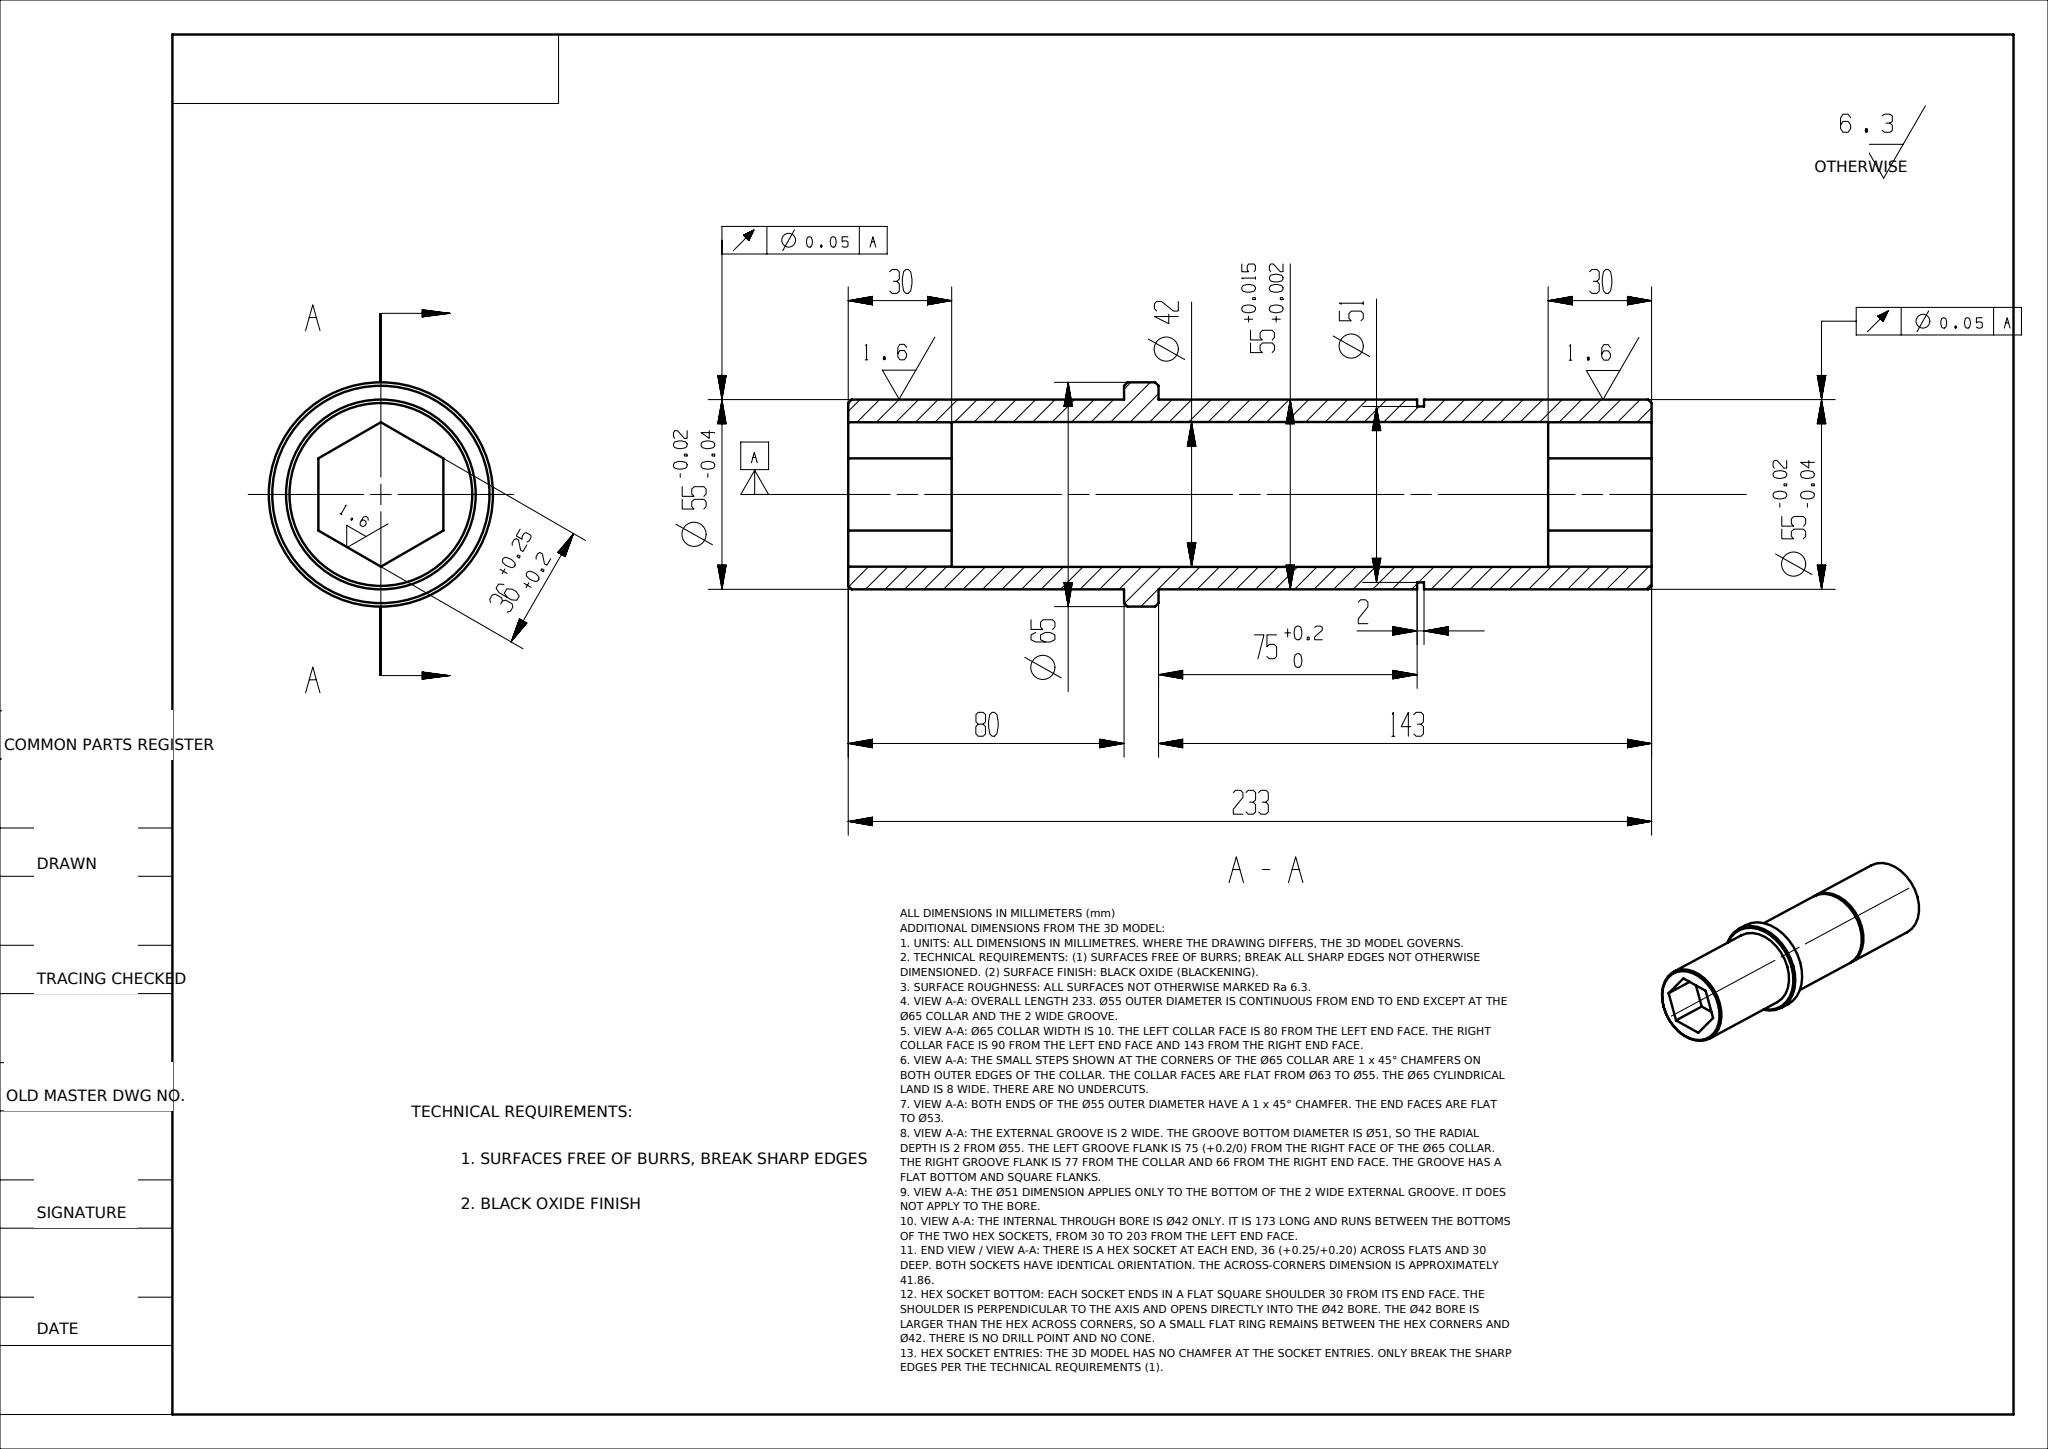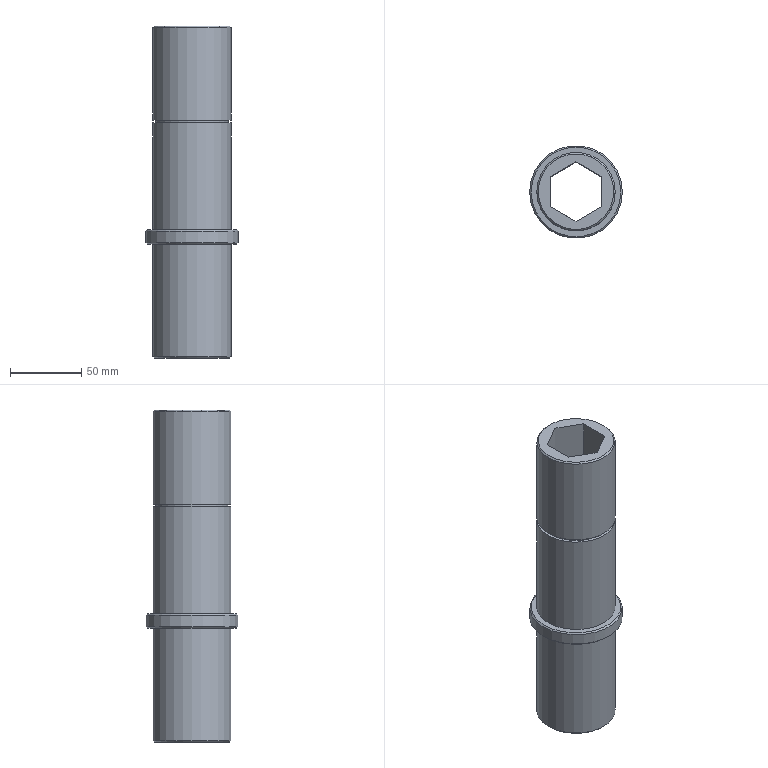Part | NX | mm | 1 solid | 30 faces | box 65 x 65 x 233 mm | volume 253992 mm3 | plane 20 | cylinder 6 | cone 4 | commonest cylinder face diameters 55 x3 65 x1 51 x1 42 x1
STEP:
#1=CARTESIAN_POINT('',(0.,0.,0.));
#2=DIRECTION('',(0.,0.,1.));
#3=DIRECTION('',(1.,0.,0.));
#4=AXIS2_PLACEMENT_3D('',#1,#2,#3);
#5=(LENGTH_UNIT()NAMED_UNIT(*)SI_UNIT(.MILLI.,.METRE.));
#6=UNCERTAINTY_MEASURE_WITH_UNIT(LENGTH_MEASURE(0.00002),#5,'','');
#7=(NAMED_UNIT(*)PLANE_ANGLE_UNIT()SI_UNIT($,.RADIAN.));
#8=PLANE_ANGLE_MEASURE_WITH_UNIT(PLANE_ANGLE_MEASURE(0.01745),#7);
#9=DIMENSIONAL_EXPONENTS(0.,0.,0.,0.,0.,0.,0.);
#10=(CONVERSION_BASED_UNIT('',#8)NAMED_UNIT(#9)PLANE_ANGLE_UNIT());
#11=(NAMED_UNIT(*)SI_UNIT($,.STERADIAN.)SOLID_ANGLE_UNIT());
#12=(GEOMETRIC_REPRESENTATION_CONTEXT(3)GLOBAL_UNCERTAINTY_ASSIGNED_CONTEXT((#6))GLOBAL_UNIT_ASSIGNED_CONTEXT((#5,#10,#11))REPRESENTATION_CONTEXT('',''));
#13=SHAPE_REPRESENTATION('',(#4),#12);
#14=CARTESIAN_POINT('',(-26.5,0.,20.));
#15=VERTEX_POINT('',#14);
#16=CARTESIAN_POINT('',(0.,0.,20.));
#17=DIRECTION('',(0.,0.,-1.));
#18=DIRECTION('',(-1.,0.,0.));
#19=AXIS2_PLACEMENT_3D('',#16,#17,#18);
#20=CIRCLE('',#19,26.5);
#21=EDGE_CURVE('',#15,#15,#20,.T.);
#22=ORIENTED_EDGE('',*,*,#21,.T.);
#23=EDGE_LOOP('',(#22));
#24=FACE_BOUND('',#23,.T.);
#25=CARTESIAN_POINT('',(-0.,20.929,20.));
#26=VERTEX_POINT('',#25);
#27=CARTESIAN_POINT('',(-18.125,10.464,20.));
#28=VERTEX_POINT('',#27);
#29=CARTESIAN_POINT('',(-9.063,15.697,20.));
#30=DIRECTION('',(-0.866,-0.5,0.));
#31=VECTOR('',#30,1.);
#32=LINE('',#29,#31);
#33=EDGE_CURVE('',#26,#28,#32,.T.);
#34=ORIENTED_EDGE('',*,*,#33,.T.);
#35=CARTESIAN_POINT('',(-18.125,-10.464,20.));
#36=VERTEX_POINT('',#35);
#37=CARTESIAN_POINT('',(-18.125,0.,20.));
#38=DIRECTION('',(0.,-1.,0.));
#39=VECTOR('',#38,1.);
#40=LINE('',#37,#39);
#41=EDGE_CURVE('',#28,#36,#40,.T.);
#42=ORIENTED_EDGE('',*,*,#41,.T.);
#43=CARTESIAN_POINT('',(0.,-20.929,20.));
#44=VERTEX_POINT('',#43);
#45=CARTESIAN_POINT('',(-9.062,-15.697,20.));
#46=DIRECTION('',(0.866,-0.5,0.));
#47=VECTOR('',#46,1.);
#48=LINE('',#45,#47);
#49=EDGE_CURVE('',#36,#44,#48,.T.);
#50=ORIENTED_EDGE('',*,*,#49,.T.);
#51=CARTESIAN_POINT('',(18.125,-10.464,20.));
#52=VERTEX_POINT('',#51);
#53=CARTESIAN_POINT('',(9.063,-15.697,20.));
#54=DIRECTION('',(0.866,0.5,0.));
#55=VECTOR('',#54,1.);
#56=LINE('',#53,#55);
#57=EDGE_CURVE('',#44,#52,#56,.T.);
#58=ORIENTED_EDGE('',*,*,#57,.T.);
#59=CARTESIAN_POINT('',(18.125,10.464,20.));
#60=VERTEX_POINT('',#59);
#61=CARTESIAN_POINT('',(18.125,0.,20.));
#62=DIRECTION('',(0.,1.,0.));
#63=VECTOR('',#62,1.);
#64=LINE('',#61,#63);
#65=EDGE_CURVE('',#52,#60,#64,.T.);
#66=ORIENTED_EDGE('',*,*,#65,.T.);
#67=CARTESIAN_POINT('',(9.062,15.697,20.));
#68=DIRECTION('',(-0.866,0.5,0.));
#69=VECTOR('',#68,1.);
#70=LINE('',#67,#69);
#71=EDGE_CURVE('',#60,#26,#70,.T.);
#72=ORIENTED_EDGE('',*,*,#71,.T.);
#73=EDGE_LOOP('',(#34,#42,#50,#58,#66,#72));
#74=FACE_BOUND('',#73,.T.);
#75=CARTESIAN_POINT('',(0.,0.,20.));
#76=DIRECTION('',(0.,0.,-1.));
#77=DIRECTION('',(-1.,0.,0.));
#78=AXIS2_PLACEMENT_3D('',#75,#76,#77);
#79=PLANE('',#78);
#80=ADVANCED_FACE('',(#24,#74),#79,.T.);
#81=CARTESIAN_POINT('',(26.5,0.,253.));
#82=VERTEX_POINT('',#81);
#83=CARTESIAN_POINT('',(0.,0.,253.));
#84=DIRECTION('',(0.,0.,1.));
#85=DIRECTION('',(1.,0.,0.));
#86=AXIS2_PLACEMENT_3D('',#83,#84,#85);
#87=CIRCLE('',#86,26.5);
#88=EDGE_CURVE('',#82,#82,#87,.T.);
#89=ORIENTED_EDGE('',*,*,#88,.T.);
#90=EDGE_LOOP('',(#89));
#91=FACE_BOUND('',#90,.T.);
#92=CARTESIAN_POINT('',(0.,-20.929,253.));
#93=VERTEX_POINT('',#92);
#94=CARTESIAN_POINT('',(-18.125,-10.464,253.));
#95=VERTEX_POINT('',#94);
#96=CARTESIAN_POINT('',(-9.062,-15.697,253.));
#97=DIRECTION('',(-0.866,0.5,0.));
#98=VECTOR('',#97,1.);
#99=LINE('',#96,#98);
#100=EDGE_CURVE('',#93,#95,#99,.T.);
#101=ORIENTED_EDGE('',*,*,#100,.T.);
#102=CARTESIAN_POINT('',(-18.125,10.464,253.));
#103=VERTEX_POINT('',#102);
#104=CARTESIAN_POINT('',(-18.125,0.,253.));
#105=DIRECTION('',(0.,1.,0.));
#106=VECTOR('',#105,1.);
#107=LINE('',#104,#106);
#108=EDGE_CURVE('',#95,#103,#107,.T.);
#109=ORIENTED_EDGE('',*,*,#108,.T.);
#110=CARTESIAN_POINT('',(-0.,20.929,253.));
#111=VERTEX_POINT('',#110);
#112=CARTESIAN_POINT('',(-9.063,15.697,253.));
#113=DIRECTION('',(0.866,0.5,0.));
#114=VECTOR('',#113,1.);
#115=LINE('',#112,#114);
#116=EDGE_CURVE('',#103,#111,#115,.T.);
#117=ORIENTED_EDGE('',*,*,#116,.T.);
#118=CARTESIAN_POINT('',(18.125,10.464,253.));
#119=VERTEX_POINT('',#118);
#120=CARTESIAN_POINT('',(9.062,15.697,253.));
#121=DIRECTION('',(0.866,-0.5,0.));
#122=VECTOR('',#121,1.);
#123=LINE('',#120,#122);
#124=EDGE_CURVE('',#111,#119,#123,.T.);
#125=ORIENTED_EDGE('',*,*,#124,.T.);
#126=CARTESIAN_POINT('',(18.125,-10.464,253.));
#127=VERTEX_POINT('',#126);
#128=CARTESIAN_POINT('',(18.125,0.,253.));
#129=DIRECTION('',(0.,-1.,0.));
#130=VECTOR('',#129,1.);
#131=LINE('',#128,#130);
#132=EDGE_CURVE('',#119,#127,#131,.T.);
#133=ORIENTED_EDGE('',*,*,#132,.T.);
#134=CARTESIAN_POINT('',(9.063,-15.697,253.));
#135=DIRECTION('',(-0.866,-0.5,0.));
#136=VECTOR('',#135,1.);
#137=LINE('',#134,#136);
#138=EDGE_CURVE('',#127,#93,#137,.T.);
#139=ORIENTED_EDGE('',*,*,#138,.T.);
#140=EDGE_LOOP('',(#101,#109,#117,#125,#133,#139));
#141=FACE_BOUND('',#140,.T.);
#142=CARTESIAN_POINT('',(0.,0.,253.));
#143=DIRECTION('',(0.,0.,1.));
#144=DIRECTION('',(1.,0.,0.));
#145=AXIS2_PLACEMENT_3D('',#142,#143,#144);
#146=PLANE('',#145);
#147=ADVANCED_FACE('',(#91,#141),#146,.T.);
#148=CARTESIAN_POINT('',(27.5,0.,110.));
#149=VERTEX_POINT('',#148);
#150=CARTESIAN_POINT('',(0.,0.,110.));
#151=DIRECTION('',(0.,0.,-1.));
#152=DIRECTION('',(1.,0.,0.));
#153=AXIS2_PLACEMENT_3D('',#150,#151,#152);
#154=CIRCLE('',#153,27.5);
#155=EDGE_CURVE('',#149,#149,#154,.T.);
#156=ORIENTED_EDGE('',*,*,#155,.F.);
#157=EDGE_LOOP('',(#156));
#158=FACE_BOUND('',#157,.T.);
#159=CARTESIAN_POINT('',(27.5,0.,185.));
#160=VERTEX_POINT('',#159);
#161=CARTESIAN_POINT('',(0.,0.,185.));
#162=DIRECTION('',(0.,0.,-1.));
#163=DIRECTION('',(1.,0.,0.));
#164=AXIS2_PLACEMENT_3D('',#161,#162,#163);
#165=CIRCLE('',#164,27.5);
#166=EDGE_CURVE('',#160,#160,#165,.T.);
#167=ORIENTED_EDGE('',*,*,#166,.T.);
#168=EDGE_LOOP('',(#167));
#169=FACE_BOUND('',#168,.T.);
#170=CARTESIAN_POINT('',(0.,0.,0.));
#171=DIRECTION('',(0.,0.,1.));
#172=DIRECTION('',(1.,0.,0.));
#173=AXIS2_PLACEMENT_3D('',#170,#171,#172);
#174=CYLINDRICAL_SURFACE('',#173,27.5);
#175=ADVANCED_FACE('',(#158,#169),#174,.T.);
#176=CARTESIAN_POINT('',(32.5,0.,109.));
#177=VERTEX_POINT('',#176);
#178=CARTESIAN_POINT('',(0.,0.,109.));
#179=DIRECTION('',(0.,0.,-1.));
#180=DIRECTION('',(1.,0.,0.));
#181=AXIS2_PLACEMENT_3D('',#178,#179,#180);
#182=CIRCLE('',#181,32.5);
#183=EDGE_CURVE('',#177,#177,#182,.T.);
#184=ORIENTED_EDGE('',*,*,#183,.T.);
#185=EDGE_LOOP('',(#184));
#186=FACE_BOUND('',#185,.T.);
#187=CARTESIAN_POINT('',(32.5,0.,101.));
#188=VERTEX_POINT('',#187);
#189=CARTESIAN_POINT('',(0.,0.,101.));
#190=DIRECTION('',(0.,0.,1.));
#191=DIRECTION('',(1.,0.,0.));
#192=AXIS2_PLACEMENT_3D('',#189,#190,#191);
#193=CIRCLE('',#192,32.5);
#194=EDGE_CURVE('',#188,#188,#193,.T.);
#195=ORIENTED_EDGE('',*,*,#194,.T.);
#196=EDGE_LOOP('',(#195));
#197=FACE_BOUND('',#196,.T.);
#198=CARTESIAN_POINT('',(0.,0.,110.));
#199=DIRECTION('',(0.,0.,-1.));
#200=DIRECTION('',(-1.,0.,0.));
#201=AXIS2_PLACEMENT_3D('',#198,#199,#200);
#202=CYLINDRICAL_SURFACE('',#201,32.5);
#203=ADVANCED_FACE('',(#186,#197),#202,.T.);
#204=CARTESIAN_POINT('',(31.5,0.,110.));
#205=VERTEX_POINT('',#204);
#206=CARTESIAN_POINT('',(0.,0.,110.));
#207=DIRECTION('',(0.,0.,1.));
#208=DIRECTION('',(1.,0.,0.));
#209=AXIS2_PLACEMENT_3D('',#206,#207,#208);
#210=CIRCLE('',#209,31.5);
#211=EDGE_CURVE('',#205,#205,#210,.T.);
#212=ORIENTED_EDGE('',*,*,#211,.T.);
#213=EDGE_LOOP('',(#212));
#214=FACE_BOUND('',#213,.T.);
#215=ORIENTED_EDGE('',*,*,#155,.T.);
#216=EDGE_LOOP('',(#215));
#217=FACE_BOUND('',#216,.T.);
#218=CARTESIAN_POINT('',(0.,0.,110.));
#219=DIRECTION('',(0.,0.,1.));
#220=DIRECTION('',(1.,0.,0.));
#221=AXIS2_PLACEMENT_3D('',#218,#219,#220);
#222=PLANE('',#221);
#223=ADVANCED_FACE('',(#214,#217),#222,.T.);
#224=CARTESIAN_POINT('',(31.5,0.,100.));
#225=VERTEX_POINT('',#224);
#226=CARTESIAN_POINT('',(0.,0.,100.));
#227=DIRECTION('',(0.,0.,-1.));
#228=DIRECTION('',(1.,0.,0.));
#229=AXIS2_PLACEMENT_3D('',#226,#227,#228);
#230=CIRCLE('',#229,31.5);
#231=EDGE_CURVE('',#225,#225,#230,.T.);
#232=ORIENTED_EDGE('',*,*,#231,.T.);
#233=EDGE_LOOP('',(#232));
#234=FACE_BOUND('',#233,.T.);
#235=CARTESIAN_POINT('',(27.5,0.,100.));
#236=VERTEX_POINT('',#235);
#237=CARTESIAN_POINT('',(0.,0.,100.));
#238=DIRECTION('',(0.,0.,-1.));
#239=DIRECTION('',(1.,0.,0.));
#240=AXIS2_PLACEMENT_3D('',#237,#238,#239);
#241=CIRCLE('',#240,27.5);
#242=EDGE_CURVE('',#236,#236,#241,.T.);
#243=ORIENTED_EDGE('',*,*,#242,.F.);
#244=EDGE_LOOP('',(#243));
#245=FACE_BOUND('',#244,.T.);
#246=CARTESIAN_POINT('',(0.,0.,100.));
#247=DIRECTION('',(0.,0.,1.));
#248=DIRECTION('',(1.,0.,0.));
#249=AXIS2_PLACEMENT_3D('',#246,#247,#248);
#250=PLANE('',#249);
#251=ADVANCED_FACE('',(#234,#245),#250,.F.);
#252=CARTESIAN_POINT('',(-27.5,0.,21.));
#253=VERTEX_POINT('',#252);
#254=CARTESIAN_POINT('',(0.,0.,21.));
#255=DIRECTION('',(0.,0.,1.));
#256=DIRECTION('',(-1.,0.,0.));
#257=AXIS2_PLACEMENT_3D('',#254,#255,#256);
#258=CIRCLE('',#257,27.5);
#259=EDGE_CURVE('',#253,#253,#258,.T.);
#260=ORIENTED_EDGE('',*,*,#259,.T.);
#261=EDGE_LOOP('',(#260));
#262=FACE_BOUND('',#261,.T.);
#263=ORIENTED_EDGE('',*,*,#242,.T.);
#264=EDGE_LOOP('',(#263));
#265=FACE_BOUND('',#264,.T.);
#266=CARTESIAN_POINT('',(0.,0.,0.));
#267=DIRECTION('',(0.,0.,1.));
#268=DIRECTION('',(1.,0.,0.));
#269=AXIS2_PLACEMENT_3D('',#266,#267,#268);
#270=CYLINDRICAL_SURFACE('',#269,27.5);
#271=ADVANCED_FACE('',(#262,#265),#270,.T.);
#272=CARTESIAN_POINT('',(25.5,0.,187.));
#273=VERTEX_POINT('',#272);
#274=CARTESIAN_POINT('',(0.,0.,187.));
#275=DIRECTION('',(0.,0.,-1.));
#276=DIRECTION('',(1.,0.,0.));
#277=AXIS2_PLACEMENT_3D('',#274,#275,#276);
#278=CIRCLE('',#277,25.5);
#279=EDGE_CURVE('',#273,#273,#278,.T.);
#280=ORIENTED_EDGE('',*,*,#279,.T.);
#281=EDGE_LOOP('',(#280));
#282=FACE_BOUND('',#281,.T.);
#283=CARTESIAN_POINT('',(25.5,0.,185.));
#284=VERTEX_POINT('',#283);
#285=CARTESIAN_POINT('',(0.,0.,185.));
#286=DIRECTION('',(0.,0.,-1.));
#287=DIRECTION('',(1.,0.,0.));
#288=AXIS2_PLACEMENT_3D('',#285,#286,#287);
#289=CIRCLE('',#288,25.5);
#290=EDGE_CURVE('',#284,#284,#289,.T.);
#291=ORIENTED_EDGE('',*,*,#290,.F.);
#292=EDGE_LOOP('',(#291));
#293=FACE_BOUND('',#292,.T.);
#294=CARTESIAN_POINT('',(0.,0.,186.));
#295=DIRECTION('',(0.,0.,1.));
#296=DIRECTION('',(1.,0.,0.));
#297=AXIS2_PLACEMENT_3D('',#294,#295,#296);
#298=CYLINDRICAL_SURFACE('',#297,25.5);
#299=ADVANCED_FACE('',(#282,#293),#298,.T.);
#300=ORIENTED_EDGE('',*,*,#166,.F.);
#301=EDGE_LOOP('',(#300));
#302=FACE_BOUND('',#301,.T.);
#303=ORIENTED_EDGE('',*,*,#290,.T.);
#304=EDGE_LOOP('',(#303));
#305=FACE_BOUND('',#304,.T.);
#306=CARTESIAN_POINT('',(0.,0.,185.));
#307=DIRECTION('',(0.,0.,1.));
#308=DIRECTION('',(1.,0.,0.));
#309=AXIS2_PLACEMENT_3D('',#306,#307,#308);
#310=PLANE('',#309);
#311=ADVANCED_FACE('',(#302,#305),#310,.T.);
#312=CARTESIAN_POINT('',(27.5,0.,187.));
#313=VERTEX_POINT('',#312);
#314=CARTESIAN_POINT('',(0.,0.,187.));
#315=DIRECTION('',(0.,0.,-1.));
#316=DIRECTION('',(1.,0.,0.));
#317=AXIS2_PLACEMENT_3D('',#314,#315,#316);
#318=CIRCLE('',#317,27.5);
#319=EDGE_CURVE('',#313,#313,#318,.T.);
#320=ORIENTED_EDGE('',*,*,#319,.T.);
#321=EDGE_LOOP('',(#320));
#322=FACE_BOUND('',#321,.T.);
#323=ORIENTED_EDGE('',*,*,#279,.F.);
#324=EDGE_LOOP('',(#323));
#325=FACE_BOUND('',#324,.T.);
#326=CARTESIAN_POINT('',(0.,0.,187.));
#327=DIRECTION('',(0.,0.,1.));
#328=DIRECTION('',(1.,0.,0.));
#329=AXIS2_PLACEMENT_3D('',#326,#327,#328);
#330=PLANE('',#329);
#331=ADVANCED_FACE('',(#322,#325),#330,.F.);
#332=CARTESIAN_POINT('',(27.5,0.,252.));
#333=VERTEX_POINT('',#332);
#334=CARTESIAN_POINT('',(0.,0.,252.));
#335=DIRECTION('',(0.,0.,-1.));
#336=DIRECTION('',(1.,0.,0.));
#337=AXIS2_PLACEMENT_3D('',#334,#335,#336);
#338=CIRCLE('',#337,27.5);
#339=EDGE_CURVE('',#333,#333,#338,.T.);
#340=ORIENTED_EDGE('',*,*,#339,.T.);
#341=EDGE_LOOP('',(#340));
#342=FACE_BOUND('',#341,.T.);
#343=ORIENTED_EDGE('',*,*,#319,.F.);
#344=EDGE_LOOP('',(#343));
#345=FACE_BOUND('',#344,.T.);
#346=CARTESIAN_POINT('',(0.,0.,0.));
#347=DIRECTION('',(0.,0.,1.));
#348=DIRECTION('',(1.,0.,0.));
#349=AXIS2_PLACEMENT_3D('',#346,#347,#348);
#350=CYLINDRICAL_SURFACE('',#349,27.5);
#351=ADVANCED_FACE('',(#342,#345),#350,.T.);
#352=ORIENTED_EDGE('',*,*,#88,.F.);
#353=EDGE_LOOP('',(#352));
#354=FACE_BOUND('',#353,.T.);
#355=ORIENTED_EDGE('',*,*,#339,.F.);
#356=EDGE_LOOP('',(#355));
#357=FACE_BOUND('',#356,.T.);
#358=CARTESIAN_POINT('',(0.,0.,252.));
#359=DIRECTION('',(0.,0.,-1.));
#360=DIRECTION('',(-1.,0.,0.));
#361=AXIS2_PLACEMENT_3D('',#358,#359,#360);
#362=CONICAL_SURFACE('',#361,27.5,45.);
#363=ADVANCED_FACE('',(#354,#357),#362,.T.);
#364=ORIENTED_EDGE('',*,*,#21,.F.);
#365=EDGE_LOOP('',(#364));
#366=FACE_BOUND('',#365,.T.);
#367=ORIENTED_EDGE('',*,*,#259,.F.);
#368=EDGE_LOOP('',(#367));
#369=FACE_BOUND('',#368,.T.);
#370=CARTESIAN_POINT('',(0.,0.,21.));
#371=DIRECTION('',(0.,0.,1.));
#372=DIRECTION('',(1.,0.,-0.));
#373=AXIS2_PLACEMENT_3D('',#370,#371,#372);
#374=CONICAL_SURFACE('',#373,27.5,45.);
#375=ADVANCED_FACE('',(#366,#369),#374,.T.);
#376=ORIENTED_EDGE('',*,*,#183,.F.);
#377=EDGE_LOOP('',(#376));
#378=FACE_BOUND('',#377,.T.);
#379=ORIENTED_EDGE('',*,*,#211,.F.);
#380=EDGE_LOOP('',(#379));
#381=FACE_BOUND('',#380,.T.);
#382=CARTESIAN_POINT('',(0.,0.,110.));
#383=DIRECTION('',(0.,0.,-1.));
#384=DIRECTION('',(-1.,0.,-0.));
#385=AXIS2_PLACEMENT_3D('',#382,#383,#384);
#386=CONICAL_SURFACE('',#385,31.5,45.);
#387=ADVANCED_FACE('',(#378,#381),#386,.T.);
#388=ORIENTED_EDGE('',*,*,#231,.F.);
#389=EDGE_LOOP('',(#388));
#390=FACE_BOUND('',#389,.T.);
#391=ORIENTED_EDGE('',*,*,#194,.F.);
#392=EDGE_LOOP('',(#391));
#393=FACE_BOUND('',#392,.T.);
#394=CARTESIAN_POINT('',(0.,0.,101.));
#395=DIRECTION('',(0.,0.,1.));
#396=DIRECTION('',(1.,0.,-0.));
#397=AXIS2_PLACEMENT_3D('',#394,#395,#396);
#398=CONICAL_SURFACE('',#397,32.5,45.);
#399=ADVANCED_FACE('',(#390,#393),#398,.T.);
#400=CARTESIAN_POINT('',(-18.125,-10.464,50.));
#401=VERTEX_POINT('',#400);
#402=CARTESIAN_POINT('',(-18.125,-10.464,-10.));
#403=DIRECTION('',(0.,0.,-1.));
#404=VECTOR('',#403,1.);
#405=LINE('',#402,#404);
#406=EDGE_CURVE('',#401,#36,#405,.T.);
#407=ORIENTED_EDGE('',*,*,#406,.F.);
#408=CARTESIAN_POINT('',(0.,-20.929,50.));
#409=VERTEX_POINT('',#408);
#410=CARTESIAN_POINT('',(-9.062,-15.697,50.));
#411=DIRECTION('',(0.866,-0.5,0.));
#412=VECTOR('',#411,1.);
#413=LINE('',#410,#412);
#414=EDGE_CURVE('',#401,#409,#413,.T.);
#415=ORIENTED_EDGE('',*,*,#414,.T.);
#416=CARTESIAN_POINT('',(0.,-20.929,-10.));
#417=DIRECTION('',(0.,0.,-1.));
#418=VECTOR('',#417,1.);
#419=LINE('',#416,#418);
#420=EDGE_CURVE('',#409,#44,#419,.T.);
#421=ORIENTED_EDGE('',*,*,#420,.T.);
#422=ORIENTED_EDGE('',*,*,#49,.F.);
#423=EDGE_LOOP('',(#407,#415,#421,#422));
#424=FACE_OUTER_BOUND('',#423,.T.);
#425=CARTESIAN_POINT('',(-0.0625,-20.893,-10.));
#426=DIRECTION('',(0.5,0.866,0.));
#427=DIRECTION('',(-0.866,0.5,0.));
#428=AXIS2_PLACEMENT_3D('',#425,#426,#427);
#429=PLANE('',#428);
#430=ADVANCED_FACE('',(#424),#429,.T.);
#431=ORIENTED_EDGE('',*,*,#420,.F.);
#432=CARTESIAN_POINT('',(18.125,-10.464,50.));
#433=VERTEX_POINT('',#432);
#434=CARTESIAN_POINT('',(9.063,-15.697,50.));
#435=DIRECTION('',(0.866,0.5,0.));
#436=VECTOR('',#435,1.);
#437=LINE('',#434,#436);
#438=EDGE_CURVE('',#409,#433,#437,.T.);
#439=ORIENTED_EDGE('',*,*,#438,.T.);
#440=CARTESIAN_POINT('',(18.125,-10.464,-10.));
#441=DIRECTION('',(0.,0.,-1.));
#442=VECTOR('',#441,1.);
#443=LINE('',#440,#442);
#444=EDGE_CURVE('',#433,#52,#443,.T.);
#445=ORIENTED_EDGE('',*,*,#444,.T.);
#446=ORIENTED_EDGE('',*,*,#57,.F.);
#447=EDGE_LOOP('',(#431,#439,#445,#446));
#448=FACE_OUTER_BOUND('',#447,.T.);
#449=CARTESIAN_POINT('',(18.062,-10.501,-10.));
#450=DIRECTION('',(-0.5,0.866,0.));
#451=DIRECTION('',(-0.866,-0.5,0.));
#452=AXIS2_PLACEMENT_3D('',#449,#450,#451);
#453=PLANE('',#452);
#454=ADVANCED_FACE('',(#448),#453,.T.);
#455=ORIENTED_EDGE('',*,*,#444,.F.);
#456=CARTESIAN_POINT('',(18.125,10.464,50.));
#457=VERTEX_POINT('',#456);
#458=CARTESIAN_POINT('',(18.125,0.,50.));
#459=DIRECTION('',(0.,1.,0.));
#460=VECTOR('',#459,1.);
#461=LINE('',#458,#460);
#462=EDGE_CURVE('',#433,#457,#461,.T.);
#463=ORIENTED_EDGE('',*,*,#462,.T.);
#464=CARTESIAN_POINT('',(18.125,10.464,-10.));
#465=DIRECTION('',(0.,0.,-1.));
#466=VECTOR('',#465,1.);
#467=LINE('',#464,#466);
#468=EDGE_CURVE('',#457,#60,#467,.T.);
#469=ORIENTED_EDGE('',*,*,#468,.T.);
#470=ORIENTED_EDGE('',*,*,#65,.F.);
#471=EDGE_LOOP('',(#455,#463,#469,#470));
#472=FACE_OUTER_BOUND('',#471,.T.);
#473=CARTESIAN_POINT('',(18.125,10.392,-10.));
#474=DIRECTION('',(-1.,0.,0.));
#475=DIRECTION('',(0.,0.,1.));
#476=AXIS2_PLACEMENT_3D('',#473,#474,#475);
#477=PLANE('',#476);
#478=ADVANCED_FACE('',(#472),#477,.T.);
#479=ORIENTED_EDGE('',*,*,#468,.F.);
#480=CARTESIAN_POINT('',(-0.,20.929,50.));
#481=VERTEX_POINT('',#480);
#482=CARTESIAN_POINT('',(9.062,15.697,50.));
#483=DIRECTION('',(-0.866,0.5,0.));
#484=VECTOR('',#483,1.);
#485=LINE('',#482,#484);
#486=EDGE_CURVE('',#457,#481,#485,.T.);
#487=ORIENTED_EDGE('',*,*,#486,.T.);
#488=CARTESIAN_POINT('',(-0.,20.929,-10.));
#489=DIRECTION('',(0.,0.,-1.));
#490=VECTOR('',#489,1.);
#491=LINE('',#488,#490);
#492=EDGE_CURVE('',#481,#26,#491,.T.);
#493=ORIENTED_EDGE('',*,*,#492,.T.);
#494=ORIENTED_EDGE('',*,*,#71,.F.);
#495=EDGE_LOOP('',(#479,#487,#493,#494));
#496=FACE_OUTER_BOUND('',#495,.T.);
#497=CARTESIAN_POINT('',(0.0625,20.893,-10.));
#498=DIRECTION('',(-0.5,-0.866,0.));
#499=DIRECTION('',(0.866,-0.5,0.));
#500=AXIS2_PLACEMENT_3D('',#497,#498,#499);
#501=PLANE('',#500);
#502=ADVANCED_FACE('',(#496),#501,.T.);
#503=ORIENTED_EDGE('',*,*,#492,.F.);
#504=CARTESIAN_POINT('',(-18.125,10.464,50.));
#505=VERTEX_POINT('',#504);
#506=CARTESIAN_POINT('',(-9.063,15.697,50.));
#507=DIRECTION('',(-0.866,-0.5,0.));
#508=VECTOR('',#507,1.);
#509=LINE('',#506,#508);
#510=EDGE_CURVE('',#481,#505,#509,.T.);
#511=ORIENTED_EDGE('',*,*,#510,.T.);
#512=CARTESIAN_POINT('',(-18.125,10.464,-10.));
#513=DIRECTION('',(0.,0.,-1.));
#514=VECTOR('',#513,1.);
#515=LINE('',#512,#514);
#516=EDGE_CURVE('',#505,#28,#515,.T.);
#517=ORIENTED_EDGE('',*,*,#516,.T.);
#518=ORIENTED_EDGE('',*,*,#33,.F.);
#519=EDGE_LOOP('',(#503,#511,#517,#518));
#520=FACE_OUTER_BOUND('',#519,.T.);
#521=CARTESIAN_POINT('',(-18.062,10.501,-10.));
#522=DIRECTION('',(0.5,-0.866,0.));
#523=DIRECTION('',(0.866,0.5,0.));
#524=AXIS2_PLACEMENT_3D('',#521,#522,#523);
#525=PLANE('',#524);
#526=ADVANCED_FACE('',(#520),#525,.T.);
#527=ORIENTED_EDGE('',*,*,#516,.F.);
#528=CARTESIAN_POINT('',(-18.125,0.,50.));
#529=DIRECTION('',(0.,-1.,0.));
#530=VECTOR('',#529,1.);
#531=LINE('',#528,#530);
#532=EDGE_CURVE('',#505,#401,#531,.T.);
#533=ORIENTED_EDGE('',*,*,#532,.T.);
#534=ORIENTED_EDGE('',*,*,#406,.T.);
#535=ORIENTED_EDGE('',*,*,#41,.F.);
#536=EDGE_LOOP('',(#527,#533,#534,#535));
#537=FACE_OUTER_BOUND('',#536,.T.);
#538=CARTESIAN_POINT('',(-18.125,-10.392,-10.));
#539=DIRECTION('',(1.,0.,0.));
#540=DIRECTION('',(0.,0.,-1.));
#541=AXIS2_PLACEMENT_3D('',#538,#539,#540);
#542=PLANE('',#541);
#543=ADVANCED_FACE('',(#537),#542,.T.);
#544=CARTESIAN_POINT('',(-18.125,-10.464,223.));
#545=VERTEX_POINT('',#544);
#546=CARTESIAN_POINT('',(-18.125,-10.464,-10.));
#547=DIRECTION('',(0.,0.,-1.));
#548=VECTOR('',#547,1.);
#549=LINE('',#546,#548);
#550=EDGE_CURVE('',#95,#545,#549,.T.);
#551=ORIENTED_EDGE('',*,*,#550,.T.);
#552=CARTESIAN_POINT('',(-18.125,10.464,223.));
#553=VERTEX_POINT('',#552);
#554=CARTESIAN_POINT('',(-18.125,0.,223.));
#555=DIRECTION('',(0.,1.,0.));
#556=VECTOR('',#555,1.);
#557=LINE('',#554,#556);
#558=EDGE_CURVE('',#545,#553,#557,.T.);
#559=ORIENTED_EDGE('',*,*,#558,.T.);
#560=CARTESIAN_POINT('',(-18.125,10.464,-10.));
#561=DIRECTION('',(0.,0.,-1.));
#562=VECTOR('',#561,1.);
#563=LINE('',#560,#562);
#564=EDGE_CURVE('',#103,#553,#563,.T.);
#565=ORIENTED_EDGE('',*,*,#564,.F.);
#566=ORIENTED_EDGE('',*,*,#108,.F.);
#567=EDGE_LOOP('',(#551,#559,#565,#566));
#568=FACE_OUTER_BOUND('',#567,.T.);
#569=CARTESIAN_POINT('',(-18.125,-10.392,-10.));
#570=DIRECTION('',(1.,0.,0.));
#571=DIRECTION('',(0.,0.,-1.));
#572=AXIS2_PLACEMENT_3D('',#569,#570,#571);
#573=PLANE('',#572);
#574=ADVANCED_FACE('',(#568),#573,.T.);
#575=ORIENTED_EDGE('',*,*,#564,.T.);
#576=CARTESIAN_POINT('',(-0.,20.929,223.));
#577=VERTEX_POINT('',#576);
#578=CARTESIAN_POINT('',(-9.063,15.697,223.));
#579=DIRECTION('',(0.866,0.5,0.));
#580=VECTOR('',#579,1.);
#581=LINE('',#578,#580);
#582=EDGE_CURVE('',#553,#577,#581,.T.);
#583=ORIENTED_EDGE('',*,*,#582,.T.);
#584=CARTESIAN_POINT('',(-0.,20.929,-10.));
#585=DIRECTION('',(0.,0.,-1.));
#586=VECTOR('',#585,1.);
#587=LINE('',#584,#586);
#588=EDGE_CURVE('',#111,#577,#587,.T.);
#589=ORIENTED_EDGE('',*,*,#588,.F.);
#590=ORIENTED_EDGE('',*,*,#116,.F.);
#591=EDGE_LOOP('',(#575,#583,#589,#590));
#592=FACE_OUTER_BOUND('',#591,.T.);
#593=CARTESIAN_POINT('',(-18.062,10.501,-10.));
#594=DIRECTION('',(0.5,-0.866,0.));
#595=DIRECTION('',(0.866,0.5,0.));
#596=AXIS2_PLACEMENT_3D('',#593,#594,#595);
#597=PLANE('',#596);
#598=ADVANCED_FACE('',(#592),#597,.T.);
#599=ORIENTED_EDGE('',*,*,#588,.T.);
#600=CARTESIAN_POINT('',(18.125,10.464,223.));
#601=VERTEX_POINT('',#600);
#602=CARTESIAN_POINT('',(9.062,15.697,223.));
#603=DIRECTION('',(0.866,-0.5,0.));
#604=VECTOR('',#603,1.);
#605=LINE('',#602,#604);
#606=EDGE_CURVE('',#577,#601,#605,.T.);
#607=ORIENTED_EDGE('',*,*,#606,.T.);
#608=CARTESIAN_POINT('',(18.125,10.464,-10.));
#609=DIRECTION('',(0.,0.,-1.));
#610=VECTOR('',#609,1.);
#611=LINE('',#608,#610);
#612=EDGE_CURVE('',#119,#601,#611,.T.);
#613=ORIENTED_EDGE('',*,*,#612,.F.);
#614=ORIENTED_EDGE('',*,*,#124,.F.);
#615=EDGE_LOOP('',(#599,#607,#613,#614));
#616=FACE_OUTER_BOUND('',#615,.T.);
#617=CARTESIAN_POINT('',(0.0625,20.893,-10.));
#618=DIRECTION('',(-0.5,-0.866,0.));
#619=DIRECTION('',(0.866,-0.5,0.));
#620=AXIS2_PLACEMENT_3D('',#617,#618,#619);
#621=PLANE('',#620);
#622=ADVANCED_FACE('',(#616),#621,.T.);
#623=ORIENTED_EDGE('',*,*,#612,.T.);
#624=CARTESIAN_POINT('',(18.125,-10.464,223.));
#625=VERTEX_POINT('',#624);
#626=CARTESIAN_POINT('',(18.125,0.,223.));
#627=DIRECTION('',(0.,-1.,0.));
#628=VECTOR('',#627,1.);
#629=LINE('',#626,#628);
#630=EDGE_CURVE('',#601,#625,#629,.T.);
#631=ORIENTED_EDGE('',*,*,#630,.T.);
#632=CARTESIAN_POINT('',(18.125,-10.464,-10.));
#633=DIRECTION('',(0.,0.,-1.));
#634=VECTOR('',#633,1.);
#635=LINE('',#632,#634);
#636=EDGE_CURVE('',#127,#625,#635,.T.);
#637=ORIENTED_EDGE('',*,*,#636,.F.);
#638=ORIENTED_EDGE('',*,*,#132,.F.);
#639=EDGE_LOOP('',(#623,#631,#637,#638));
#640=FACE_OUTER_BOUND('',#639,.T.);
#641=CARTESIAN_POINT('',(18.125,10.392,-10.));
#642=DIRECTION('',(-1.,0.,0.));
#643=DIRECTION('',(0.,0.,1.));
#644=AXIS2_PLACEMENT_3D('',#641,#642,#643);
#645=PLANE('',#644);
#646=ADVANCED_FACE('',(#640),#645,.T.);
#647=ORIENTED_EDGE('',*,*,#636,.T.);
#648=CARTESIAN_POINT('',(0.,-20.929,223.));
#649=VERTEX_POINT('',#648);
#650=CARTESIAN_POINT('',(9.063,-15.697,223.));
#651=DIRECTION('',(-0.866,-0.5,0.));
#652=VECTOR('',#651,1.);
#653=LINE('',#650,#652);
#654=EDGE_CURVE('',#625,#649,#653,.T.);
#655=ORIENTED_EDGE('',*,*,#654,.T.);
#656=CARTESIAN_POINT('',(0.,-20.929,-10.));
#657=DIRECTION('',(0.,0.,-1.));
#658=VECTOR('',#657,1.);
#659=LINE('',#656,#658);
#660=EDGE_CURVE('',#93,#649,#659,.T.);
#661=ORIENTED_EDGE('',*,*,#660,.F.);
#662=ORIENTED_EDGE('',*,*,#138,.F.);
#663=EDGE_LOOP('',(#647,#655,#661,#662));
#664=FACE_OUTER_BOUND('',#663,.T.);
#665=CARTESIAN_POINT('',(18.062,-10.501,-10.));
#666=DIRECTION('',(-0.5,0.866,0.));
#667=DIRECTION('',(-0.866,-0.5,0.));
#668=AXIS2_PLACEMENT_3D('',#665,#666,#667);
#669=PLANE('',#668);
#670=ADVANCED_FACE('',(#664),#669,.T.);
#671=ORIENTED_EDGE('',*,*,#660,.T.);
#672=CARTESIAN_POINT('',(-9.062,-15.697,223.));
#673=DIRECTION('',(-0.866,0.5,0.));
#674=VECTOR('',#673,1.);
#675=LINE('',#672,#674);
#676=EDGE_CURVE('',#649,#545,#675,.T.);
#677=ORIENTED_EDGE('',*,*,#676,.T.);
#678=ORIENTED_EDGE('',*,*,#550,.F.);
#679=ORIENTED_EDGE('',*,*,#100,.F.);
#680=EDGE_LOOP('',(#671,#677,#678,#679));
#681=FACE_OUTER_BOUND('',#680,.T.);
#682=CARTESIAN_POINT('',(-0.0625,-20.893,-10.));
#683=DIRECTION('',(0.5,0.866,0.));
#684=DIRECTION('',(-0.866,0.5,0.));
#685=AXIS2_PLACEMENT_3D('',#682,#683,#684);
#686=PLANE('',#685);
#687=ADVANCED_FACE('',(#681),#686,.T.);
#688=CARTESIAN_POINT('',(21.,0.,223.));
#689=VERTEX_POINT('',#688);
#690=CARTESIAN_POINT('',(0.,0.,223.));
#691=DIRECTION('',(0.,0.,1.));
#692=DIRECTION('',(1.,0.,0.));
#693=AXIS2_PLACEMENT_3D('',#690,#691,#692);
#694=CIRCLE('',#693,21.);
#695=EDGE_CURVE('',#689,#689,#694,.T.);
#696=ORIENTED_EDGE('',*,*,#695,.F.);
#697=EDGE_LOOP('',(#696));
#698=FACE_BOUND('',#697,.T.);
#699=ORIENTED_EDGE('',*,*,#558,.F.);
#700=ORIENTED_EDGE('',*,*,#676,.F.);
#701=ORIENTED_EDGE('',*,*,#654,.F.);
#702=ORIENTED_EDGE('',*,*,#630,.F.);
#703=ORIENTED_EDGE('',*,*,#606,.F.);
#704=ORIENTED_EDGE('',*,*,#582,.F.);
#705=EDGE_LOOP('',(#699,#700,#701,#702,#703,#704));
#706=FACE_BOUND('',#705,.T.);
#707=CARTESIAN_POINT('',(0.,0.,223.));
#708=DIRECTION('',(0.,0.,1.));
#709=DIRECTION('',(1.,0.,0.));
#710=AXIS2_PLACEMENT_3D('',#707,#708,#709);
#711=PLANE('',#710);
#712=ADVANCED_FACE('',(#698,#706),#711,.F.);
#713=CARTESIAN_POINT('',(-21.,0.,50.));
#714=VERTEX_POINT('',#713);
#715=CARTESIAN_POINT('',(0.,0.,50.));
#716=DIRECTION('',(0.,0.,-1.));
#717=DIRECTION('',(-1.,0.,0.));
#718=AXIS2_PLACEMENT_3D('',#715,#716,#717);
#719=CIRCLE('',#718,21.);
#720=EDGE_CURVE('',#714,#714,#719,.T.);
#721=ORIENTED_EDGE('',*,*,#720,.F.);
#722=EDGE_LOOP('',(#721));
#723=FACE_BOUND('',#722,.T.);
#724=ORIENTED_EDGE('',*,*,#532,.F.);
#725=ORIENTED_EDGE('',*,*,#510,.F.);
#726=ORIENTED_EDGE('',*,*,#486,.F.);
#727=ORIENTED_EDGE('',*,*,#462,.F.);
#728=ORIENTED_EDGE('',*,*,#438,.F.);
#729=ORIENTED_EDGE('',*,*,#414,.F.);
#730=EDGE_LOOP('',(#724,#725,#726,#727,#728,#729));
#731=FACE_BOUND('',#730,.T.);
#732=CARTESIAN_POINT('',(0.,0.,50.));
#733=DIRECTION('',(0.,0.,-1.));
#734=DIRECTION('',(-1.,0.,0.));
#735=AXIS2_PLACEMENT_3D('',#732,#733,#734);
#736=PLANE('',#735);
#737=ADVANCED_FACE('',(#723,#731),#736,.F.);
#738=ORIENTED_EDGE('',*,*,#695,.T.);
#739=EDGE_LOOP('',(#738));
#740=FACE_BOUND('',#739,.T.);
#741=ORIENTED_EDGE('',*,*,#720,.T.);
#742=EDGE_LOOP('',(#741));
#743=FACE_BOUND('',#742,.T.);
#744=CARTESIAN_POINT('',(0.,0.,0.));
#745=DIRECTION('',(0.,0.,1.));
#746=DIRECTION('',(1.,0.,0.));
#747=AXIS2_PLACEMENT_3D('',#744,#745,#746);
#748=CYLINDRICAL_SURFACE('',#747,21.);
#749=ADVANCED_FACE('',(#740,#743),#748,.F.);
#750=CLOSED_SHELL('',(#80,#147,#175,#203,#223,#251,#271,#299,#311,#331,#351,#363,#375,#387,#399,#430,#454,#478,#502,#526,#543,#574,#598,#622,#646,#670,#687,#712,#737,#749));
#751=MANIFOLD_SOLID_BREP('',#750);
#752=ADVANCED_BREP_SHAPE_REPRESENTATION('',(#751),#12);
#753=SHAPE_REPRESENTATION_RELATIONSHIP('','',#13,#752);
#754=PRESENTATION_LAYER_ASSIGNMENT('','',(#751));
#755=COLOUR_RGB('',0.4902,0.4902,0.4902);
#756=FILL_AREA_STYLE_COLOUR('',#755);
#757=FILL_AREA_STYLE('',(#756));
#758=SURFACE_STYLE_FILL_AREA(#757);
#759=SURFACE_SIDE_STYLE('',(#758));
#760=SURFACE_STYLE_USAGE(.BOTH.,#759);
#761=PRESENTATION_STYLE_ASSIGNMENT((#760));
#762=STYLED_ITEM('',(#761),#751);
#763=MECHANICAL_DESIGN_GEOMETRIC_PRESENTATION_REPRESENTATION('',(#762),#12);